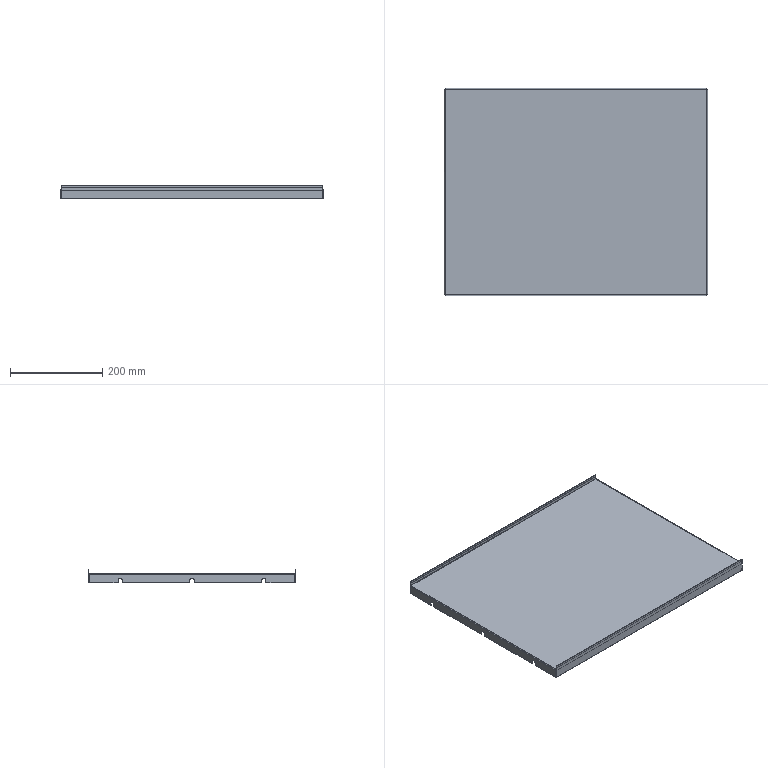Component | SolidWorks | Shelf-1 | 1 solid | 100 faces | volume 265479 mm3 | plane 64 | cylinder 28 | spline 8 | commonest cylinder face diameters 9 x12 3.6 x4 2 x4 1.7 x4 0.1 x4 | material 304